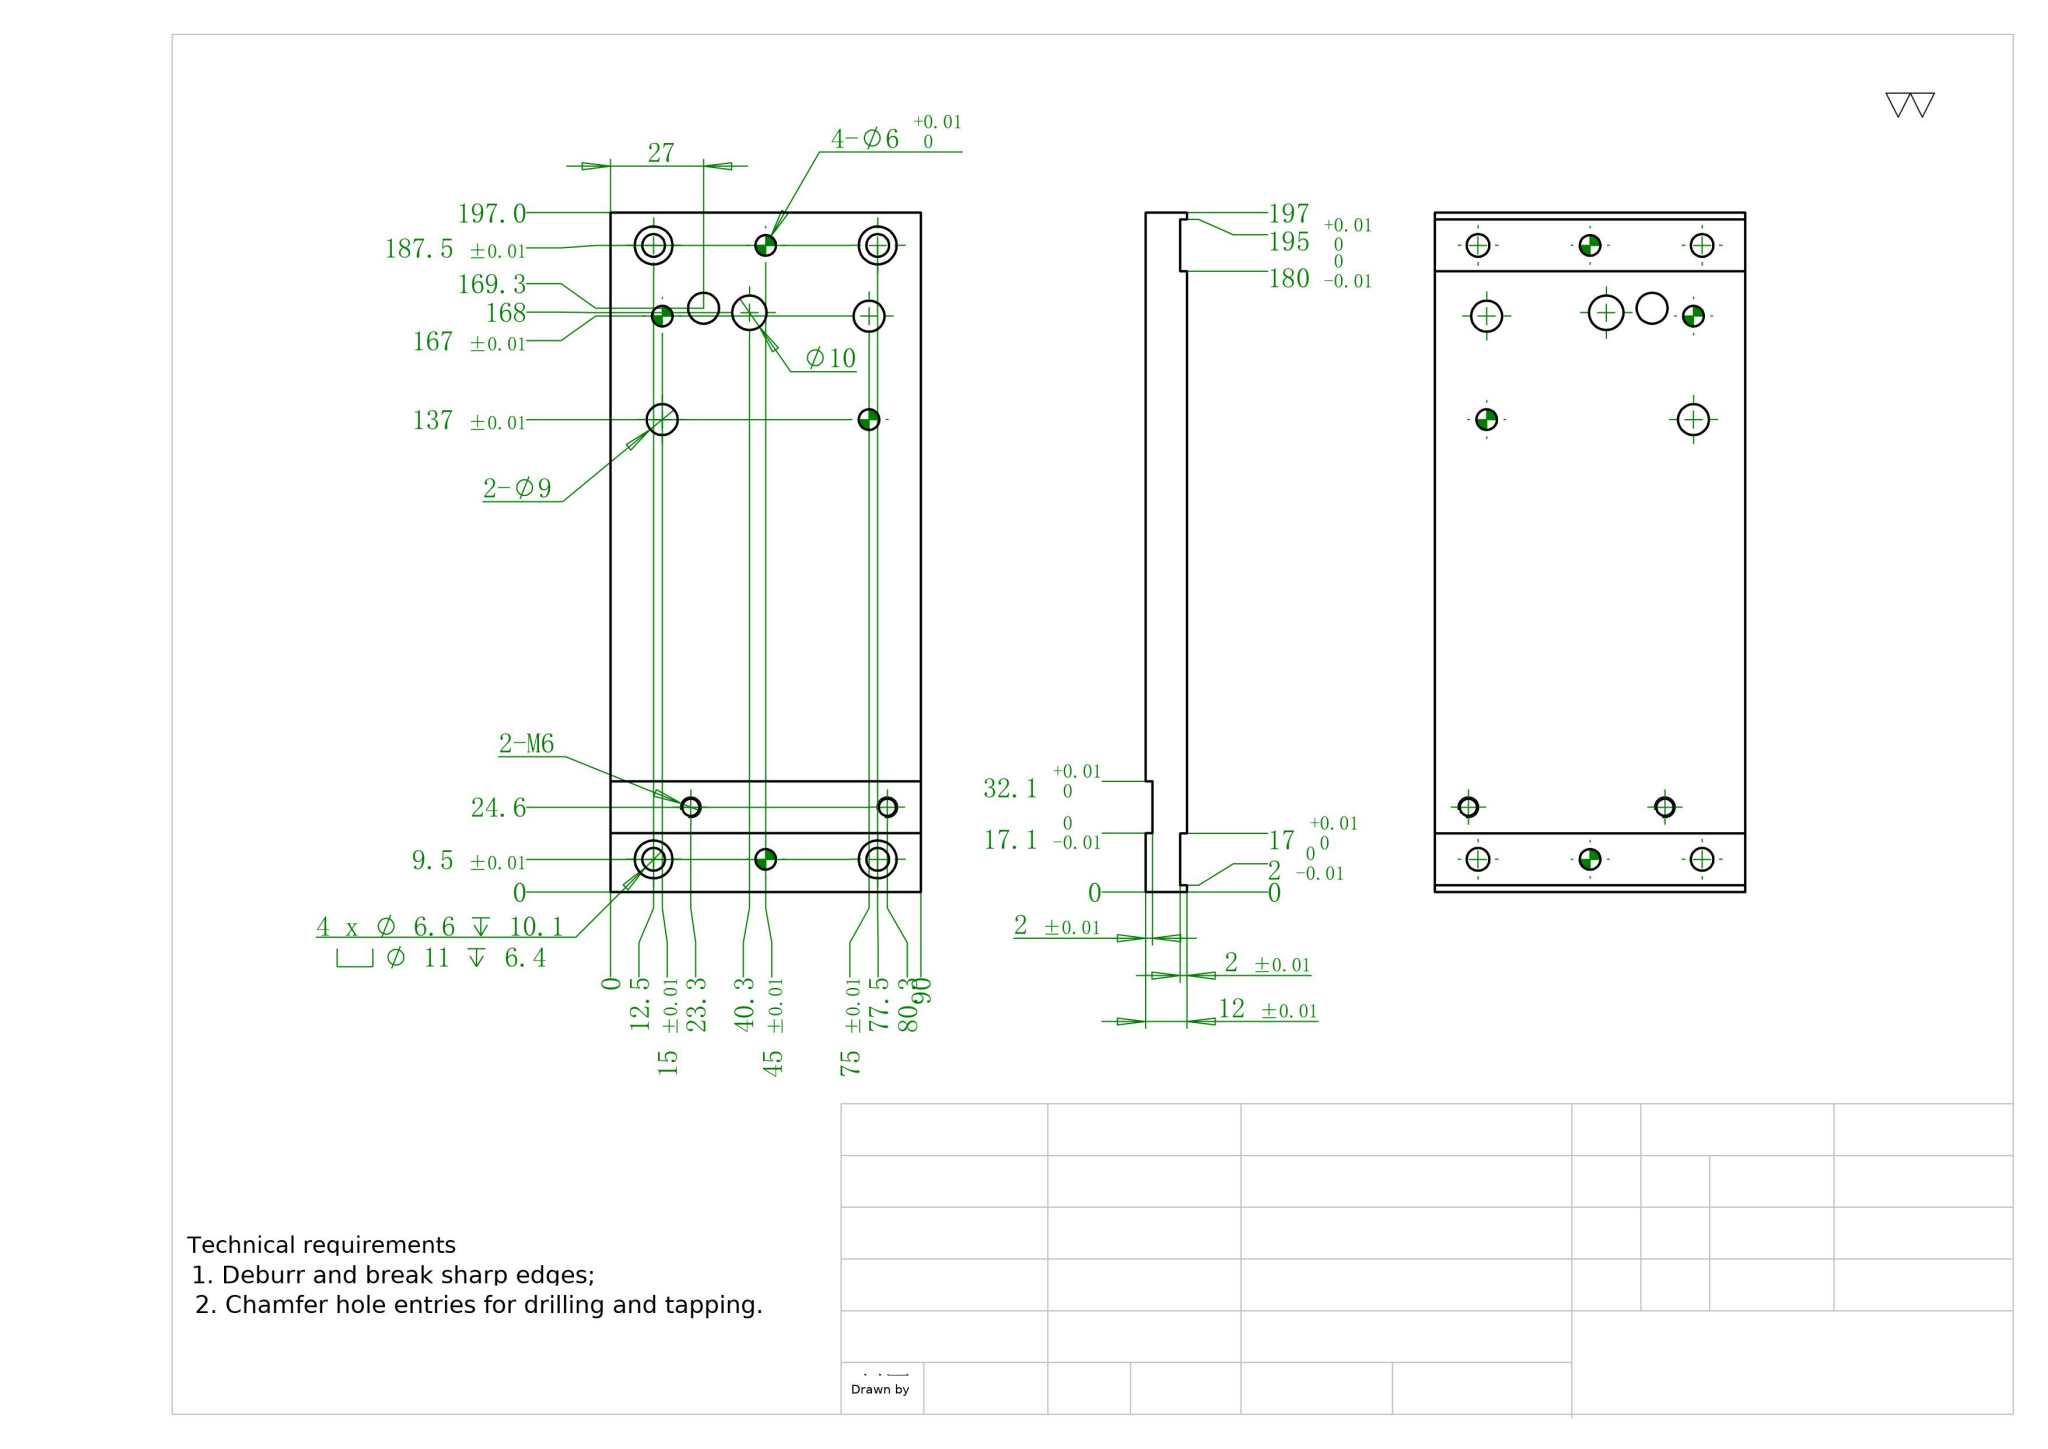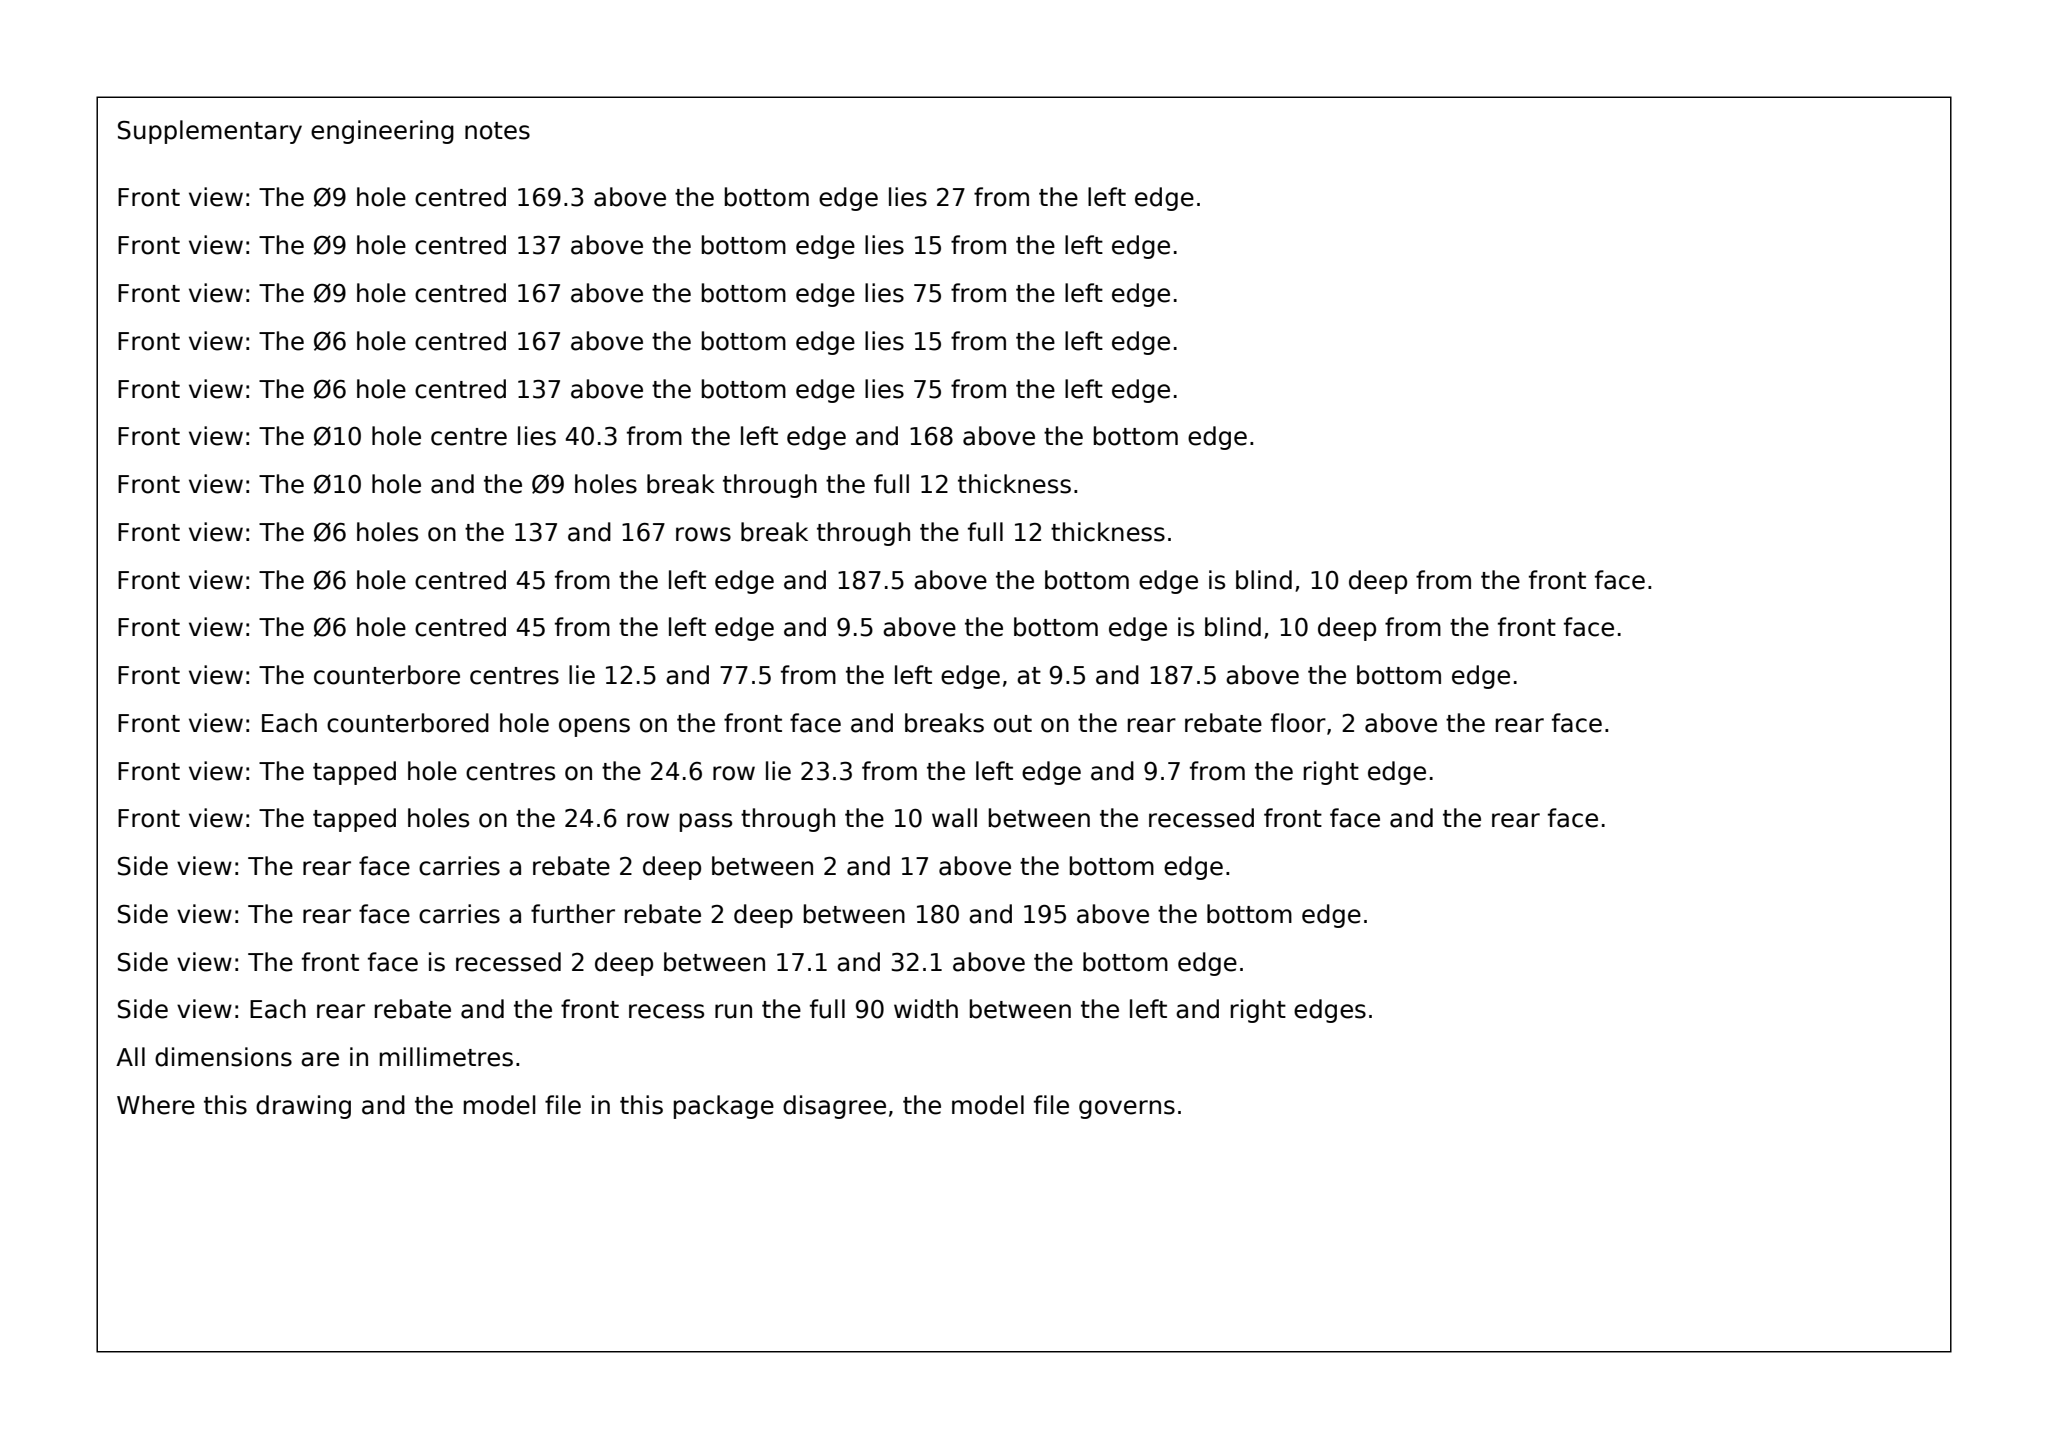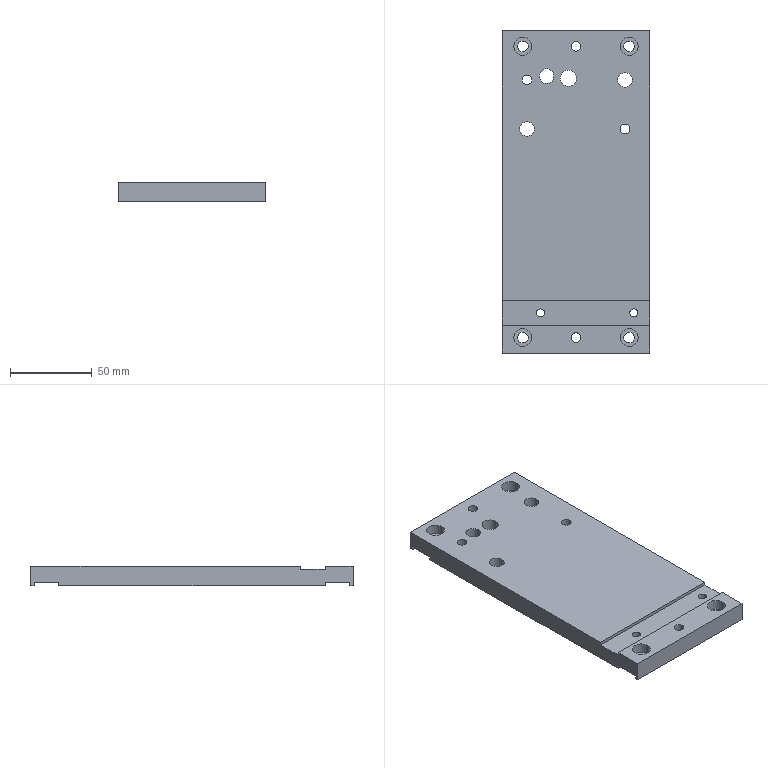Part | SolidWorks | mm | 1 solid | 58 faces | box 90 x 197 x 12 mm | volume 196865 mm3 | cylinder 36 | plane 22 | commonest cylinder face diameters 6 x8 11 x8 6.6 x8 9 x6 5 x4 10 x2
Drawing notes:
2-Ø6 +0.01/0 DP 10 BLIND AT X45/Y9.5 & X45/Y187.5; OTHER 2 THRU | from the solid: Ø6 cyl len 10 at (45,9.5) & (45,187.5); Ø6 len 12 (=plate thk) at (15,167) & (75,137)
2-M6 DP 10, DRILL Ø5 DP 10 (BLIND) | from the solid: Ø5 z-cyl len 10 at (23.3,24.6) and (80.3,24.6); plate thk 12
CHANGE TO 3-Ø9 THRU; 3RD HOLE AT X27, Y169.3 | from the solid: Ø9 z-cyl len 12 (thru) at (15,137), (75,167), (27,169.3)
build123d program:
from build123d import *

# Parameters (mm, degrees)
SKETCH1_W                                       = 90
SKETCH1_H                                       = 12
BOSS_EXTRUDE1_DEPTH                             = 197
SKETCH2_W                                       = 2
SKETCH2_H                                       = 15
CUT_EXTRUDE1_DEPTH                              = 217.668
SKETCH3_W                                       = 2
SKETCH3_H                                       = 15
CUT_EXTRUDE2_DEPTH                              = 217.668
M6_HEX_SOCKET_HEAD_CAP_SCREW_CBORE1_D           = 6.6
M6_HEX_SOCKET_HEAD_CAP_SCREW_CBORE1_DEPTH       = 10.1
M6_HEX_SOCKET_HEAD_CAP_SCREW_CBORE1_CBORE_D     = 11
M6_HEX_SOCKET_HEAD_CAP_SCREW_CBORE1_CBORE_DEPTH = 6.4
M6_HEX_SOCKET_HEAD_CAP_SCREW_CBORE1_TIP         = 1.983
F_6_0_6_DIAMETER_HOLE2_D                        = 6
SKETCH9_R                                       = 5
CUT_EXTRUDE3_DEPTH                              = 203.43
M6_TAPPED_HOLE1_D                               = 5
SKETCH12_W                                      = 2
SKETCH12_H                                      = 15
CUT_EXTRUDE4_DEPTH                              = 217.668
F_9_0_9_DIAMETER_HOLE1_D                        = 9
F_9_0_9_DIAMETER_HOLE1_DEPTH                    = 15
F_9_0_9_DIAMETER_HOLE1_TIP                      = 2.704
F_6_0_6_DIAMETER_HOLE3_D                        = 6
F_6_0_6_DIAMETER_HOLE3_DEPTH                    = 15
F_6_0_6_DIAMETER_HOLE3_TIP                      = 1.803
SKETCH17_R                                      = 4.5
CUT_EXTRUDE5_DEPTH                              = 203.43


with BuildPart() as part:
    # Sketch1 → Boss-Extrude1 (new body)
    with BuildSketch(Plane(origin=(0, 0, 0), x_dir=(1, 0, 0), z_dir=(0, 1, 0))):
        Rectangle(SKETCH1_W, SKETCH1_H)
    extrude(amount=BOSS_EXTRUDE1_DEPTH)

    # Sketch2 → Cut-Extrude1 (cut, through all)
    with BuildSketch(Plane(origin=(45, 0, 0), x_dir=(0, 0, -1), z_dir=(1, 0, 0))):
        with Locations((5, 187.5)):
            Rectangle(SKETCH2_W, SKETCH2_H)
    extrude(amount=-CUT_EXTRUDE1_DEPTH, mode=Mode.SUBTRACT)

    # Sketch3 → Cut-Extrude2 (cut, through all)
    with BuildSketch(Plane(origin=(45, 0, 0), x_dir=(0, 0, -1), z_dir=(1, 0, 0))):
        with Locations((5, 9.5)):
            Rectangle(SKETCH3_W, SKETCH3_H)
    extrude(amount=-CUT_EXTRUDE2_DEPTH, mode=Mode.SUBTRACT)

    # M6 Hex Socket Head Cap Screw CBORE1
    with Locations(Plane.XY.offset(6)):
        with Locations((-32.5, 187.5), (32.5, 187.5), (32.5, 9.5), (-32.5, 9.5)):
            CounterBoreHole(M6_HEX_SOCKET_HEAD_CAP_SCREW_CBORE1_D / 2, M6_HEX_SOCKET_HEAD_CAP_SCREW_CBORE1_CBORE_D / 2, M6_HEX_SOCKET_HEAD_CAP_SCREW_CBORE1_CBORE_DEPTH, depth=M6_HEX_SOCKET_HEAD_CAP_SCREW_CBORE1_DEPTH)
            with Locations((0, 0, -(M6_HEX_SOCKET_HEAD_CAP_SCREW_CBORE1_DEPTH + M6_HEX_SOCKET_HEAD_CAP_SCREW_CBORE1_TIP / 2))):  # 118° drill point
                Cone(0, M6_HEX_SOCKET_HEAD_CAP_SCREW_CBORE1_D / 2, M6_HEX_SOCKET_HEAD_CAP_SCREW_CBORE1_TIP, mode=Mode.SUBTRACT)

    # 6.0 _6_ Diameter Hole2 (through all)
    with Locations(Plane.XY.offset(6)):
        with Locations((0, 187.5), (0, 9.5)):
            Hole(F_6_0_6_DIAMETER_HOLE2_D / 2)

    # Sketch9 → Cut-Extrude3 (cut, through all)
    with BuildSketch(Plane(origin=(0, 0, -6), x_dir=(-1, 0, 0), z_dir=(0, 0, -1))):
        with Locations((4.7, 168)):
            Circle(SKETCH9_R)
    extrude(amount=-CUT_EXTRUDE3_DEPTH, mode=Mode.SUBTRACT)

    # M6 Tapped Hole1 (through all)
    with Locations(Plane.XY.offset(6)):
        with Locations((35.3, 24.6), (-21.7, 24.6)):
            Hole(M6_TAPPED_HOLE1_D / 2)

    # Sketch12 → Cut-Extrude4 (cut, through all)
    with BuildSketch(Plane.ZY.offset(45)):
        with Locations((5, 24.6)):
            Rectangle(SKETCH12_W, SKETCH12_H)
    extrude(amount=-CUT_EXTRUDE4_DEPTH, mode=Mode.SUBTRACT)

    # 9.0 _9_ Diameter Hole1
    with Locations(Plane(origin=(0, 0, -6), x_dir=(-1, 0, 0), z_dir=(0, 0, -1))):
        with Locations((-30, 167), (30, 137)):
            Hole(F_9_0_9_DIAMETER_HOLE1_D / 2, depth=F_9_0_9_DIAMETER_HOLE1_DEPTH)
            with Locations((0, 0, -(F_9_0_9_DIAMETER_HOLE1_DEPTH + F_9_0_9_DIAMETER_HOLE1_TIP / 2))):  # 118° drill point
                Cone(0, F_9_0_9_DIAMETER_HOLE1_D / 2, F_9_0_9_DIAMETER_HOLE1_TIP, mode=Mode.SUBTRACT)

    # 6.0 _6_ Diameter Hole3
    with Locations(Plane(origin=(0, 0, -6), x_dir=(-1, 0, 0), z_dir=(0, 0, -1))):
        with Locations((30, 167), (-30, 137)):
            Hole(F_6_0_6_DIAMETER_HOLE3_D / 2, depth=F_6_0_6_DIAMETER_HOLE3_DEPTH)
            with Locations((0, 0, -(F_6_0_6_DIAMETER_HOLE3_DEPTH + F_6_0_6_DIAMETER_HOLE3_TIP / 2))):  # 118° drill point
                Cone(0, F_6_0_6_DIAMETER_HOLE3_D / 2, F_6_0_6_DIAMETER_HOLE3_TIP, mode=Mode.SUBTRACT)

    # Sketch17 → Cut-Extrude5 (cut, through all)
    with BuildSketch(Plane.XY.offset(6)):
        with Locations((-18, 169.3)):
            Circle(SKETCH17_R)
    extrude(amount=-CUT_EXTRUDE5_DEPTH, mode=Mode.SUBTRACT)


solid = part.part